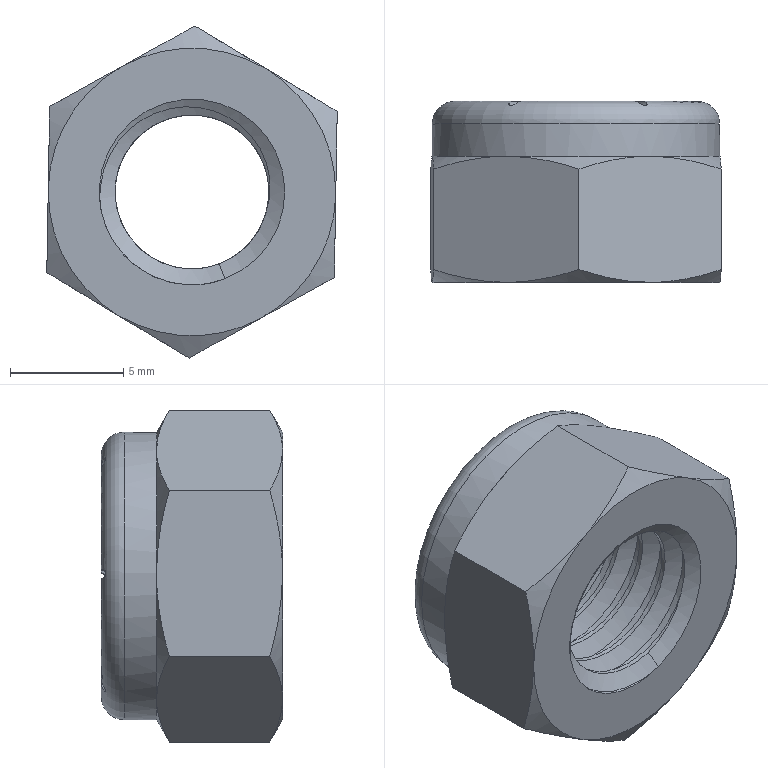Component | NX | HANGERAXLENUT_2 | 1 solid | 48 faces | volume 707 mm3 | plane 19 | cone 15 | cylinder 10 | spline 3 | torus 1 | commonest cylinder face diameters 0.4 x6 8.211 x2 12.7 x1 6.8 x1